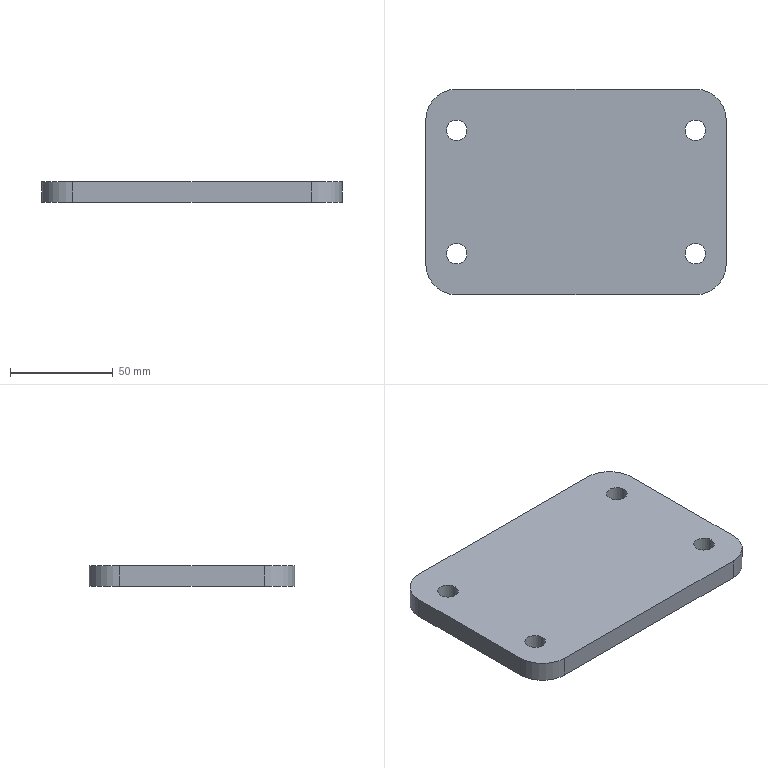Component | NX | BASE_100 | 1 solid | 14 faces | box 146 x 100 x 10 mm | volume 140927 mm3 | cylinder 8 | plane 6 | commonest cylinder face diameters 10 x4 30 x4
STEP:
#1=CARTESIAN_POINT('',(0.,0.,0.));
#2=DIRECTION('',(0.,0.,1.));
#3=DIRECTION('',(1.,0.,0.));
#4=AXIS2_PLACEMENT_3D('',#1,#2,#3);
#5=CARTESIAN_POINT('',(-73.,-35.,50.));
#6=VERTEX_POINT('',#5);
#7=CARTESIAN_POINT('',(-73.,35.,50.));
#8=VERTEX_POINT('',#7);
#9=CARTESIAN_POINT('',(-73.,-50.,50.));
#10=DIRECTION('',(0.,1.,0.));
#11=VECTOR('',#10,1.);
#12=LINE('',#9,#11);
#13=CARTESIAN_POINT('',(-73.,-50.,50.));
#14=DIRECTION('',(1.,0.,0.));
#15=DIRECTION('',(0.,0.,1.));
#16=AXIS2_PLACEMENT_3D('',#13,#14,#15);
#17=PLANE('',#16);
#18=CARTESIAN_POINT('',(0.,0.));
#19=DIRECTION('',(0.,-1.));
#20=VECTOR('',#19,1.);
#21=LINE('',#18,#20);
#22=(GEOMETRIC_REPRESENTATION_CONTEXT(2)PARAMETRIC_REPRESENTATION_CONTEXT()REPRESENTATION_CONTEXT('',''));
#23=DEFINITIONAL_REPRESENTATION('',(#21),#22);
#24=PCURVE('',#17,#23);
#25=CARTESIAN_POINT('',(-58.,30.,50.));
#26=DIRECTION('',(0.,0.,-1.));
#27=DIRECTION('',(1.,0.,0.));
#28=AXIS2_PLACEMENT_3D('',#25,#26,#27);
#29=PLANE('',#28);
#30=CARTESIAN_POINT('',(-15.,80.));
#31=DIRECTION('',(0.,-1.));
#32=VECTOR('',#31,1.);
#33=LINE('',#30,#32);
#34=(GEOMETRIC_REPRESENTATION_CONTEXT(2)PARAMETRIC_REPRESENTATION_CONTEXT()REPRESENTATION_CONTEXT('',''));
#35=DEFINITIONAL_REPRESENTATION('',(#33),#34);
#36=PCURVE('',#29,#35);
#37=SURFACE_CURVE('',#12,(#24,#36),.PCURVE_S1.);
#38=EDGE_CURVE('',#6,#8,#37,.T.);
#39=ORIENTED_EDGE('',*,*,#38,.F.);
#40=CARTESIAN_POINT('',(-73.,-35.,60.));
#41=VERTEX_POINT('',#40);
#42=CARTESIAN_POINT('',(-73.,-35.,50.));
#43=DIRECTION('',(0.,0.,1.));
#44=VECTOR('',#43,1.);
#45=LINE('',#42,#44);
#46=CARTESIAN_POINT('',(0.,-15.));
#47=DIRECTION('',(1.,0.));
#48=VECTOR('',#47,1.);
#49=LINE('',#46,#48);
#50=(GEOMETRIC_REPRESENTATION_CONTEXT(2)PARAMETRIC_REPRESENTATION_CONTEXT()REPRESENTATION_CONTEXT('',''));
#51=DEFINITIONAL_REPRESENTATION('',(#49),#50);
#52=PCURVE('',#17,#51);
#53=CARTESIAN_POINT('',(-58.,-35.,50.));
#54=DIRECTION('',(0.,0.,1.));
#55=DIRECTION('',(-1.,0.,0.));
#56=AXIS2_PLACEMENT_3D('',#53,#54,#55);
#57=CYLINDRICAL_SURFACE('',#56,15.);
#58=CARTESIAN_POINT('',(0.,0.));
#59=DIRECTION('',(0.,1.));
#60=VECTOR('',#59,1.);
#61=LINE('',#58,#60);
#62=(GEOMETRIC_REPRESENTATION_CONTEXT(2)PARAMETRIC_REPRESENTATION_CONTEXT()REPRESENTATION_CONTEXT('',''));
#63=DEFINITIONAL_REPRESENTATION('',(#61),#62);
#64=PCURVE('',#57,#63);
#65=SURFACE_CURVE('',#45,(#52,#64),.PCURVE_S1.);
#66=EDGE_CURVE('',#6,#41,#65,.T.);
#67=ORIENTED_EDGE('',*,*,#66,.T.);
#68=CARTESIAN_POINT('',(-73.,35.,60.));
#69=VERTEX_POINT('',#68);
#70=CARTESIAN_POINT('',(-73.,-50.,60.));
#71=DIRECTION('',(0.,1.,0.));
#72=VECTOR('',#71,1.);
#73=LINE('',#70,#72);
#74=CARTESIAN_POINT('',(10.,0.));
#75=DIRECTION('',(0.,-1.));
#76=VECTOR('',#75,1.);
#77=LINE('',#74,#76);
#78=(GEOMETRIC_REPRESENTATION_CONTEXT(2)PARAMETRIC_REPRESENTATION_CONTEXT()REPRESENTATION_CONTEXT('',''));
#79=DEFINITIONAL_REPRESENTATION('',(#77),#78);
#80=PCURVE('',#17,#79);
#81=CARTESIAN_POINT('',(-58.,30.,60.));
#82=DIRECTION('',(0.,0.,-1.));
#83=DIRECTION('',(1.,0.,0.));
#84=AXIS2_PLACEMENT_3D('',#81,#82,#83);
#85=PLANE('',#84);
#86=CARTESIAN_POINT('',(-15.,80.));
#87=DIRECTION('',(0.,-1.));
#88=VECTOR('',#87,1.);
#89=LINE('',#86,#88);
#90=(GEOMETRIC_REPRESENTATION_CONTEXT(2)PARAMETRIC_REPRESENTATION_CONTEXT()REPRESENTATION_CONTEXT('',''));
#91=DEFINITIONAL_REPRESENTATION('',(#89),#90);
#92=PCURVE('',#85,#91);
#93=SURFACE_CURVE('',#73,(#80,#92),.PCURVE_S1.);
#94=EDGE_CURVE('',#41,#69,#93,.T.);
#95=ORIENTED_EDGE('',*,*,#94,.T.);
#96=CARTESIAN_POINT('',(-73.,35.,50.));
#97=DIRECTION('',(0.,0.,-1.));
#98=VECTOR('',#97,1.);
#99=LINE('',#96,#98);
#100=CARTESIAN_POINT('',(0.,-85.));
#101=DIRECTION('',(-1.,0.));
#102=VECTOR('',#101,1.);
#103=LINE('',#100,#102);
#104=(GEOMETRIC_REPRESENTATION_CONTEXT(2)PARAMETRIC_REPRESENTATION_CONTEXT()REPRESENTATION_CONTEXT('',''));
#105=DEFINITIONAL_REPRESENTATION('',(#103),#104);
#106=PCURVE('',#17,#105);
#107=CARTESIAN_POINT('',(-58.,35.,50.));
#108=DIRECTION('',(0.,0.,1.));
#109=DIRECTION('',(-1.,0.,0.));
#110=AXIS2_PLACEMENT_3D('',#107,#108,#109);
#111=CYLINDRICAL_SURFACE('',#110,15.);
#112=CARTESIAN_POINT('',(6.283,0.));
#113=DIRECTION('',(0.,-1.));
#114=VECTOR('',#113,1.);
#115=LINE('',#112,#114);
#116=(GEOMETRIC_REPRESENTATION_CONTEXT(2)PARAMETRIC_REPRESENTATION_CONTEXT()REPRESENTATION_CONTEXT('',''));
#117=DEFINITIONAL_REPRESENTATION('',(#115),#116);
#118=PCURVE('',#111,#117);
#119=SURFACE_CURVE('',#99,(#106,#118),.PCURVE_S1.);
#120=EDGE_CURVE('',#69,#8,#119,.T.);
#121=ORIENTED_EDGE('',*,*,#120,.T.);
#122=EDGE_LOOP('',(#39,#67,#95,#121));
#123=FACE_BOUND('',#122,.T.);
#124=ADVANCED_FACE('',(#123),#17,.F.);
#125=CARTESIAN_POINT('',(-58.,50.,60.));
#126=VERTEX_POINT('',#125);
#127=CARTESIAN_POINT('',(58.,50.,60.));
#128=VERTEX_POINT('',#127);
#129=CARTESIAN_POINT('',(-73.,50.,60.));
#130=DIRECTION('',(1.,0.,0.));
#131=VECTOR('',#130,1.);
#132=LINE('',#129,#131);
#133=CARTESIAN_POINT('',(-73.,50.,50.));
#134=DIRECTION('',(0.,-1.,0.));
#135=DIRECTION('',(-1.,-0.,0.));
#136=AXIS2_PLACEMENT_3D('',#133,#134,#135);
#137=PLANE('',#136);
#138=CARTESIAN_POINT('',(0.,-10.));
#139=DIRECTION('',(-1.,0.));
#140=VECTOR('',#139,1.);
#141=LINE('',#138,#140);
#142=(GEOMETRIC_REPRESENTATION_CONTEXT(2)PARAMETRIC_REPRESENTATION_CONTEXT()REPRESENTATION_CONTEXT('',''));
#143=DEFINITIONAL_REPRESENTATION('',(#141),#142);
#144=PCURVE('',#137,#143);
#145=CARTESIAN_POINT('',(-15.,-20.));
#146=DIRECTION('',(1.,-0.));
#147=VECTOR('',#146,1.);
#148=LINE('',#145,#147);
#149=(GEOMETRIC_REPRESENTATION_CONTEXT(2)PARAMETRIC_REPRESENTATION_CONTEXT()REPRESENTATION_CONTEXT('',''));
#150=DEFINITIONAL_REPRESENTATION('',(#148),#149);
#151=PCURVE('',#85,#150);
#152=SURFACE_CURVE('',#132,(#144,#151),.PCURVE_S1.);
#153=EDGE_CURVE('',#126,#128,#152,.T.);
#154=ORIENTED_EDGE('',*,*,#153,.T.);
#155=CARTESIAN_POINT('',(58.,50.,50.));
#156=VERTEX_POINT('',#155);
#157=CARTESIAN_POINT('',(58.,50.,50.));
#158=DIRECTION('',(0.,0.,-1.));
#159=VECTOR('',#158,1.);
#160=LINE('',#157,#159);
#161=CARTESIAN_POINT('',(-131.,0.));
#162=DIRECTION('',(0.,1.));
#163=VECTOR('',#162,1.);
#164=LINE('',#161,#163);
#165=(GEOMETRIC_REPRESENTATION_CONTEXT(2)PARAMETRIC_REPRESENTATION_CONTEXT()REPRESENTATION_CONTEXT('',''));
#166=DEFINITIONAL_REPRESENTATION('',(#164),#165);
#167=PCURVE('',#137,#166);
#168=CARTESIAN_POINT('',(58.,35.,50.));
#169=DIRECTION('',(0.,0.,1.));
#170=DIRECTION('',(-1.,0.,0.));
#171=AXIS2_PLACEMENT_3D('',#168,#169,#170);
#172=CYLINDRICAL_SURFACE('',#171,15.);
#173=CARTESIAN_POINT('',(4.712,0.));
#174=DIRECTION('',(0.,-1.));
#175=VECTOR('',#174,1.);
#176=LINE('',#173,#175);
#177=(GEOMETRIC_REPRESENTATION_CONTEXT(2)PARAMETRIC_REPRESENTATION_CONTEXT()REPRESENTATION_CONTEXT('',''));
#178=DEFINITIONAL_REPRESENTATION('',(#176),#177);
#179=PCURVE('',#172,#178);
#180=SURFACE_CURVE('',#160,(#167,#179),.PCURVE_S1.);
#181=EDGE_CURVE('',#128,#156,#180,.T.);
#182=ORIENTED_EDGE('',*,*,#181,.T.);
#183=CARTESIAN_POINT('',(-58.,50.,50.));
#184=VERTEX_POINT('',#183);
#185=CARTESIAN_POINT('',(-73.,50.,50.));
#186=DIRECTION('',(1.,0.,0.));
#187=VECTOR('',#186,1.);
#188=LINE('',#185,#187);
#189=CARTESIAN_POINT('',(0.,0.));
#190=DIRECTION('',(-1.,0.));
#191=VECTOR('',#190,1.);
#192=LINE('',#189,#191);
#193=(GEOMETRIC_REPRESENTATION_CONTEXT(2)PARAMETRIC_REPRESENTATION_CONTEXT()REPRESENTATION_CONTEXT('',''));
#194=DEFINITIONAL_REPRESENTATION('',(#192),#193);
#195=PCURVE('',#137,#194);
#196=CARTESIAN_POINT('',(-15.,-20.));
#197=DIRECTION('',(1.,-0.));
#198=VECTOR('',#197,1.);
#199=LINE('',#196,#198);
#200=(GEOMETRIC_REPRESENTATION_CONTEXT(2)PARAMETRIC_REPRESENTATION_CONTEXT()REPRESENTATION_CONTEXT('',''));
#201=DEFINITIONAL_REPRESENTATION('',(#199),#200);
#202=PCURVE('',#29,#201);
#203=SURFACE_CURVE('',#188,(#195,#202),.PCURVE_S1.);
#204=EDGE_CURVE('',#184,#156,#203,.T.);
#205=ORIENTED_EDGE('',*,*,#204,.F.);
#206=CARTESIAN_POINT('',(-58.,50.,50.));
#207=DIRECTION('',(0.,0.,1.));
#208=VECTOR('',#207,1.);
#209=LINE('',#206,#208);
#210=CARTESIAN_POINT('',(-15.,0.));
#211=DIRECTION('',(0.,-1.));
#212=VECTOR('',#211,1.);
#213=LINE('',#210,#212);
#214=(GEOMETRIC_REPRESENTATION_CONTEXT(2)PARAMETRIC_REPRESENTATION_CONTEXT()REPRESENTATION_CONTEXT('',''));
#215=DEFINITIONAL_REPRESENTATION('',(#213),#214);
#216=PCURVE('',#137,#215);
#217=CARTESIAN_POINT('',(4.712,0.));
#218=DIRECTION('',(0.,1.));
#219=VECTOR('',#218,1.);
#220=LINE('',#217,#219);
#221=(GEOMETRIC_REPRESENTATION_CONTEXT(2)PARAMETRIC_REPRESENTATION_CONTEXT()REPRESENTATION_CONTEXT('',''));
#222=DEFINITIONAL_REPRESENTATION('',(#220),#221);
#223=PCURVE('',#111,#222);
#224=SURFACE_CURVE('',#209,(#216,#223),.PCURVE_S1.);
#225=EDGE_CURVE('',#184,#126,#224,.T.);
#226=ORIENTED_EDGE('',*,*,#225,.T.);
#227=EDGE_LOOP('',(#154,#182,#205,#226));
#228=FACE_BOUND('',#227,.T.);
#229=ADVANCED_FACE('',(#228),#137,.F.);
#230=CARTESIAN_POINT('',(73.,35.,60.));
#231=VERTEX_POINT('',#230);
#232=CARTESIAN_POINT('',(73.,-35.,60.));
#233=VERTEX_POINT('',#232);
#234=CARTESIAN_POINT('',(73.,50.,60.));
#235=DIRECTION('',(0.,-1.,0.));
#236=VECTOR('',#235,1.);
#237=LINE('',#234,#236);
#238=CARTESIAN_POINT('',(73.,50.,50.));
#239=DIRECTION('',(-1.,-0.,0.));
#240=DIRECTION('',(-0.,1.,0.));
#241=AXIS2_PLACEMENT_3D('',#238,#239,#240);
#242=PLANE('',#241);
#243=CARTESIAN_POINT('',(0.,-10.));
#244=DIRECTION('',(-1.,0.));
#245=VECTOR('',#244,1.);
#246=LINE('',#243,#245);
#247=(GEOMETRIC_REPRESENTATION_CONTEXT(2)PARAMETRIC_REPRESENTATION_CONTEXT()REPRESENTATION_CONTEXT('',''));
#248=DEFINITIONAL_REPRESENTATION('',(#246),#247);
#249=PCURVE('',#242,#248);
#250=CARTESIAN_POINT('',(131.,-20.));
#251=DIRECTION('',(0.,1.));
#252=VECTOR('',#251,1.);
#253=LINE('',#250,#252);
#254=(GEOMETRIC_REPRESENTATION_CONTEXT(2)PARAMETRIC_REPRESENTATION_CONTEXT()REPRESENTATION_CONTEXT('',''));
#255=DEFINITIONAL_REPRESENTATION('',(#253),#254);
#256=PCURVE('',#85,#255);
#257=SURFACE_CURVE('',#237,(#249,#256),.PCURVE_S1.);
#258=EDGE_CURVE('',#231,#233,#257,.T.);
#259=ORIENTED_EDGE('',*,*,#258,.T.);
#260=CARTESIAN_POINT('',(73.,-35.,50.));
#261=VERTEX_POINT('',#260);
#262=CARTESIAN_POINT('',(73.,-35.,50.));
#263=DIRECTION('',(0.,0.,-1.));
#264=VECTOR('',#263,1.);
#265=LINE('',#262,#264);
#266=CARTESIAN_POINT('',(-85.,0.));
#267=DIRECTION('',(0.,1.));
#268=VECTOR('',#267,1.);
#269=LINE('',#266,#268);
#270=(GEOMETRIC_REPRESENTATION_CONTEXT(2)PARAMETRIC_REPRESENTATION_CONTEXT()REPRESENTATION_CONTEXT('',''));
#271=DEFINITIONAL_REPRESENTATION('',(#269),#270);
#272=PCURVE('',#242,#271);
#273=CARTESIAN_POINT('',(58.,-35.,50.));
#274=DIRECTION('',(0.,0.,1.));
#275=DIRECTION('',(-1.,0.,0.));
#276=AXIS2_PLACEMENT_3D('',#273,#274,#275);
#277=CYLINDRICAL_SURFACE('',#276,15.);
#278=CARTESIAN_POINT('',(3.142,0.));
#279=DIRECTION('',(0.,-1.));
#280=VECTOR('',#279,1.);
#281=LINE('',#278,#280);
#282=(GEOMETRIC_REPRESENTATION_CONTEXT(2)PARAMETRIC_REPRESENTATION_CONTEXT()REPRESENTATION_CONTEXT('',''));
#283=DEFINITIONAL_REPRESENTATION('',(#281),#282);
#284=PCURVE('',#277,#283);
#285=SURFACE_CURVE('',#265,(#272,#284),.PCURVE_S1.);
#286=EDGE_CURVE('',#233,#261,#285,.T.);
#287=ORIENTED_EDGE('',*,*,#286,.T.);
#288=CARTESIAN_POINT('',(73.,35.,50.));
#289=VERTEX_POINT('',#288);
#290=CARTESIAN_POINT('',(73.,50.,50.));
#291=DIRECTION('',(0.,-1.,0.));
#292=VECTOR('',#291,1.);
#293=LINE('',#290,#292);
#294=CARTESIAN_POINT('',(0.,0.));
#295=DIRECTION('',(-1.,0.));
#296=VECTOR('',#295,1.);
#297=LINE('',#294,#296);
#298=(GEOMETRIC_REPRESENTATION_CONTEXT(2)PARAMETRIC_REPRESENTATION_CONTEXT()REPRESENTATION_CONTEXT('',''));
#299=DEFINITIONAL_REPRESENTATION('',(#297),#298);
#300=PCURVE('',#242,#299);
#301=CARTESIAN_POINT('',(131.,-20.));
#302=DIRECTION('',(0.,1.));
#303=VECTOR('',#302,1.);
#304=LINE('',#301,#303);
#305=(GEOMETRIC_REPRESENTATION_CONTEXT(2)PARAMETRIC_REPRESENTATION_CONTEXT()REPRESENTATION_CONTEXT('',''));
#306=DEFINITIONAL_REPRESENTATION('',(#304),#305);
#307=PCURVE('',#29,#306);
#308=SURFACE_CURVE('',#293,(#300,#307),.PCURVE_S1.);
#309=EDGE_CURVE('',#289,#261,#308,.T.);
#310=ORIENTED_EDGE('',*,*,#309,.F.);
#311=CARTESIAN_POINT('',(73.,35.,50.));
#312=DIRECTION('',(0.,0.,1.));
#313=VECTOR('',#312,1.);
#314=LINE('',#311,#313);
#315=CARTESIAN_POINT('',(-15.,0.));
#316=DIRECTION('',(0.,-1.));
#317=VECTOR('',#316,1.);
#318=LINE('',#315,#317);
#319=(GEOMETRIC_REPRESENTATION_CONTEXT(2)PARAMETRIC_REPRESENTATION_CONTEXT()REPRESENTATION_CONTEXT('',''));
#320=DEFINITIONAL_REPRESENTATION('',(#318),#319);
#321=PCURVE('',#242,#320);
#322=CARTESIAN_POINT('',(3.142,0.));
#323=DIRECTION('',(0.,1.));
#324=VECTOR('',#323,1.);
#325=LINE('',#322,#324);
#326=(GEOMETRIC_REPRESENTATION_CONTEXT(2)PARAMETRIC_REPRESENTATION_CONTEXT()REPRESENTATION_CONTEXT('',''));
#327=DEFINITIONAL_REPRESENTATION('',(#325),#326);
#328=PCURVE('',#172,#327);
#329=SURFACE_CURVE('',#314,(#321,#328),.PCURVE_S1.);
#330=EDGE_CURVE('',#289,#231,#329,.T.);
#331=ORIENTED_EDGE('',*,*,#330,.T.);
#332=EDGE_LOOP('',(#259,#287,#310,#331));
#333=FACE_BOUND('',#332,.T.);
#334=ADVANCED_FACE('',(#333),#242,.F.);
#335=CARTESIAN_POINT('',(63.,30.,50.));
#336=VERTEX_POINT('',#335);
#337=CARTESIAN_POINT('',(58.,30.,50.));
#338=DIRECTION('',(0.,0.,-1.));
#339=DIRECTION('',(1.,0.,0.));
#340=AXIS2_PLACEMENT_3D('',#337,#338,#339);
#341=CIRCLE('',#340,5.);
#342=CARTESIAN_POINT('',(58.,30.,50.));
#343=DIRECTION('',(0.,0.,1.));
#344=DIRECTION('',(-1.,0.,0.));
#345=AXIS2_PLACEMENT_3D('',#342,#343,#344);
#346=CYLINDRICAL_SURFACE('',#345,5.);
#347=CARTESIAN_POINT('',(9.425,0.));
#348=DIRECTION('',(-1.,0.));
#349=VECTOR('',#348,1.);
#350=LINE('',#347,#349);
#351=(GEOMETRIC_REPRESENTATION_CONTEXT(2)PARAMETRIC_REPRESENTATION_CONTEXT()REPRESENTATION_CONTEXT('',''));
#352=DEFINITIONAL_REPRESENTATION('',(#350),#351);
#353=PCURVE('',#346,#352);
#354=CARTESIAN_POINT('',(116.,0.));
#355=DIRECTION('',(1.,0.));
#356=AXIS2_PLACEMENT_2D('',#354,#355);
#357=CIRCLE('',#356,5.);
#358=(GEOMETRIC_REPRESENTATION_CONTEXT(2)PARAMETRIC_REPRESENTATION_CONTEXT()REPRESENTATION_CONTEXT('',''));
#359=DEFINITIONAL_REPRESENTATION('',(#357),#358);
#360=PCURVE('',#29,#359);
#361=SURFACE_CURVE('',#341,(#353,#360),.PCURVE_S1.);
#362=EDGE_CURVE('',#336,#336,#361,.T.);
#363=ORIENTED_EDGE('',*,*,#362,.F.);
#364=CARTESIAN_POINT('',(63.,30.,60.));
#365=VERTEX_POINT('',#364);
#366=CARTESIAN_POINT('',(63.,30.,50.));
#367=CARTESIAN_POINT('',(63.,30.,60.));
#368=B_SPLINE_CURVE_WITH_KNOTS('',1,(#366,#367),.UNSPECIFIED.,.F.,.F.,(2,2),(0.,10.),.PIECEWISE_BEZIER_KNOTS.);
#369=CARTESIAN_POINT('',(9.425,0.));
#370=DIRECTION('',(0.,1.));
#371=VECTOR('',#370,1.);
#372=LINE('',#369,#371);
#373=(GEOMETRIC_REPRESENTATION_CONTEXT(2)PARAMETRIC_REPRESENTATION_CONTEXT()REPRESENTATION_CONTEXT('',''));
#374=DEFINITIONAL_REPRESENTATION('',(#372),#373);
#375=PCURVE('',#346,#374);
#376=CARTESIAN_POINT('',(3.142,0.));
#377=DIRECTION('',(0.,1.));
#378=VECTOR('',#377,1.);
#379=LINE('',#376,#378);
#380=(GEOMETRIC_REPRESENTATION_CONTEXT(2)PARAMETRIC_REPRESENTATION_CONTEXT()REPRESENTATION_CONTEXT('',''));
#381=DEFINITIONAL_REPRESENTATION('',(#379),#380);
#382=PCURVE('',#346,#381);
#383=SEAM_CURVE('',#368,(#375,#382),.PCURVE_S1.);
#384=EDGE_CURVE('',#336,#365,#383,.T.);
#385=ORIENTED_EDGE('',*,*,#384,.T.);
#386=CARTESIAN_POINT('',(58.,30.,60.));
#387=DIRECTION('',(0.,0.,-1.));
#388=DIRECTION('',(1.,0.,0.));
#389=AXIS2_PLACEMENT_3D('',#386,#387,#388);
#390=CIRCLE('',#389,5.);
#391=CARTESIAN_POINT('',(9.425,10.));
#392=DIRECTION('',(-1.,0.));
#393=VECTOR('',#392,1.);
#394=LINE('',#391,#393);
#395=(GEOMETRIC_REPRESENTATION_CONTEXT(2)PARAMETRIC_REPRESENTATION_CONTEXT()REPRESENTATION_CONTEXT('',''));
#396=DEFINITIONAL_REPRESENTATION('',(#394),#395);
#397=PCURVE('',#346,#396);
#398=CARTESIAN_POINT('',(116.,0.));
#399=DIRECTION('',(1.,0.));
#400=AXIS2_PLACEMENT_2D('',#398,#399);
#401=CIRCLE('',#400,5.);
#402=(GEOMETRIC_REPRESENTATION_CONTEXT(2)PARAMETRIC_REPRESENTATION_CONTEXT()REPRESENTATION_CONTEXT('',''));
#403=DEFINITIONAL_REPRESENTATION('',(#401),#402);
#404=PCURVE('',#85,#403);
#405=SURFACE_CURVE('',#390,(#397,#404),.PCURVE_S1.);
#406=EDGE_CURVE('',#365,#365,#405,.T.);
#407=ORIENTED_EDGE('',*,*,#406,.T.);
#408=ORIENTED_EDGE('',*,*,#384,.F.);
#409=EDGE_LOOP('',(#363,#385,#407,#408));
#410=FACE_BOUND('',#409,.F.);
#411=ADVANCED_FACE('',(#410),#346,.F.);
#412=CARTESIAN_POINT('',(-53.,-30.,50.));
#413=VERTEX_POINT('',#412);
#414=CARTESIAN_POINT('',(-58.,-30.,50.));
#415=DIRECTION('',(0.,0.,-1.));
#416=DIRECTION('',(1.,0.,0.));
#417=AXIS2_PLACEMENT_3D('',#414,#415,#416);
#418=CIRCLE('',#417,5.);
#419=CARTESIAN_POINT('',(-58.,-30.,50.));
#420=DIRECTION('',(0.,0.,1.));
#421=DIRECTION('',(-1.,0.,0.));
#422=AXIS2_PLACEMENT_3D('',#419,#420,#421);
#423=CYLINDRICAL_SURFACE('',#422,5.);
#424=CARTESIAN_POINT('',(9.425,0.));
#425=DIRECTION('',(-1.,0.));
#426=VECTOR('',#425,1.);
#427=LINE('',#424,#426);
#428=(GEOMETRIC_REPRESENTATION_CONTEXT(2)PARAMETRIC_REPRESENTATION_CONTEXT()REPRESENTATION_CONTEXT('',''));
#429=DEFINITIONAL_REPRESENTATION('',(#427),#428);
#430=PCURVE('',#423,#429);
#431=CARTESIAN_POINT('',(0.,60.));
#432=DIRECTION('',(1.,0.));
#433=AXIS2_PLACEMENT_2D('',#431,#432);
#434=CIRCLE('',#433,5.);
#435=(GEOMETRIC_REPRESENTATION_CONTEXT(2)PARAMETRIC_REPRESENTATION_CONTEXT()REPRESENTATION_CONTEXT('',''));
#436=DEFINITIONAL_REPRESENTATION('',(#434),#435);
#437=PCURVE('',#29,#436);
#438=SURFACE_CURVE('',#418,(#430,#437),.PCURVE_S1.);
#439=EDGE_CURVE('',#413,#413,#438,.T.);
#440=ORIENTED_EDGE('',*,*,#439,.F.);
#441=CARTESIAN_POINT('',(-53.,-30.,60.));
#442=VERTEX_POINT('',#441);
#443=CARTESIAN_POINT('',(-53.,-30.,50.));
#444=CARTESIAN_POINT('',(-53.,-30.,60.));
#445=B_SPLINE_CURVE_WITH_KNOTS('',1,(#443,#444),.UNSPECIFIED.,.F.,.F.,(2,2),(0.,10.),.PIECEWISE_BEZIER_KNOTS.);
#446=CARTESIAN_POINT('',(9.425,0.));
#447=DIRECTION('',(0.,1.));
#448=VECTOR('',#447,1.);
#449=LINE('',#446,#448);
#450=(GEOMETRIC_REPRESENTATION_CONTEXT(2)PARAMETRIC_REPRESENTATION_CONTEXT()REPRESENTATION_CONTEXT('',''));
#451=DEFINITIONAL_REPRESENTATION('',(#449),#450);
#452=PCURVE('',#423,#451);
#453=CARTESIAN_POINT('',(3.142,0.));
#454=DIRECTION('',(0.,1.));
#455=VECTOR('',#454,1.);
#456=LINE('',#453,#455);
#457=(GEOMETRIC_REPRESENTATION_CONTEXT(2)PARAMETRIC_REPRESENTATION_CONTEXT()REPRESENTATION_CONTEXT('',''));
#458=DEFINITIONAL_REPRESENTATION('',(#456),#457);
#459=PCURVE('',#423,#458);
#460=SEAM_CURVE('',#445,(#452,#459),.PCURVE_S1.);
#461=EDGE_CURVE('',#413,#442,#460,.T.);
#462=ORIENTED_EDGE('',*,*,#461,.T.);
#463=CARTESIAN_POINT('',(-58.,-30.,60.));
#464=DIRECTION('',(0.,0.,-1.));
#465=DIRECTION('',(1.,0.,0.));
#466=AXIS2_PLACEMENT_3D('',#463,#464,#465);
#467=CIRCLE('',#466,5.);
#468=CARTESIAN_POINT('',(9.425,10.));
#469=DIRECTION('',(-1.,0.));
#470=VECTOR('',#469,1.);
#471=LINE('',#468,#470);
#472=(GEOMETRIC_REPRESENTATION_CONTEXT(2)PARAMETRIC_REPRESENTATION_CONTEXT()REPRESENTATION_CONTEXT('',''));
#473=DEFINITIONAL_REPRESENTATION('',(#471),#472);
#474=PCURVE('',#423,#473);
#475=CARTESIAN_POINT('',(0.,60.));
#476=DIRECTION('',(1.,0.));
#477=AXIS2_PLACEMENT_2D('',#475,#476);
#478=CIRCLE('',#477,5.);
#479=(GEOMETRIC_REPRESENTATION_CONTEXT(2)PARAMETRIC_REPRESENTATION_CONTEXT()REPRESENTATION_CONTEXT('',''));
#480=DEFINITIONAL_REPRESENTATION('',(#478),#479);
#481=PCURVE('',#85,#480);
#482=SURFACE_CURVE('',#467,(#474,#481),.PCURVE_S1.);
#483=EDGE_CURVE('',#442,#442,#482,.T.);
#484=ORIENTED_EDGE('',*,*,#483,.T.);
#485=ORIENTED_EDGE('',*,*,#461,.F.);
#486=EDGE_LOOP('',(#440,#462,#484,#485));
#487=FACE_BOUND('',#486,.F.);
#488=ADVANCED_FACE('',(#487),#423,.F.);
#489=CARTESIAN_POINT('',(-53.,30.,50.));
#490=VERTEX_POINT('',#489);
#491=CARTESIAN_POINT('',(-58.,30.,50.));
#492=DIRECTION('',(0.,0.,-1.));
#493=DIRECTION('',(1.,0.,0.));
#494=AXIS2_PLACEMENT_3D('',#491,#492,#493);
#495=CIRCLE('',#494,5.);
#496=CARTESIAN_POINT('',(-58.,30.,50.));
#497=DIRECTION('',(0.,0.,1.));
#498=DIRECTION('',(-1.,0.,0.));
#499=AXIS2_PLACEMENT_3D('',#496,#497,#498);
#500=CYLINDRICAL_SURFACE('',#499,5.);
#501=CARTESIAN_POINT('',(9.425,0.));
#502=DIRECTION('',(-1.,0.));
#503=VECTOR('',#502,1.);
#504=LINE('',#501,#503);
#505=(GEOMETRIC_REPRESENTATION_CONTEXT(2)PARAMETRIC_REPRESENTATION_CONTEXT()REPRESENTATION_CONTEXT('',''));
#506=DEFINITIONAL_REPRESENTATION('',(#504),#505);
#507=PCURVE('',#500,#506);
#508=CARTESIAN_POINT('',(0.,0.));
#509=DIRECTION('',(1.,0.));
#510=AXIS2_PLACEMENT_2D('',#508,#509);
#511=CIRCLE('',#510,5.);
#512=(GEOMETRIC_REPRESENTATION_CONTEXT(2)PARAMETRIC_REPRESENTATION_CONTEXT()REPRESENTATION_CONTEXT('',''));
#513=DEFINITIONAL_REPRESENTATION('',(#511),#512);
#514=PCURVE('',#29,#513);
#515=SURFACE_CURVE('',#495,(#507,#514),.PCURVE_S1.);
#516=EDGE_CURVE('',#490,#490,#515,.T.);
#517=ORIENTED_EDGE('',*,*,#516,.F.);
#518=CARTESIAN_POINT('',(-53.,30.,60.));
#519=VERTEX_POINT('',#518);
#520=CARTESIAN_POINT('',(-53.,30.,50.));
#521=CARTESIAN_POINT('',(-53.,30.,60.));
#522=B_SPLINE_CURVE_WITH_KNOTS('',1,(#520,#521),.UNSPECIFIED.,.F.,.F.,(2,2),(0.,10.),.PIECEWISE_BEZIER_KNOTS.);
#523=CARTESIAN_POINT('',(9.425,0.));
#524=DIRECTION('',(0.,1.));
#525=VECTOR('',#524,1.);
#526=LINE('',#523,#525);
#527=(GEOMETRIC_REPRESENTATION_CONTEXT(2)PARAMETRIC_REPRESENTATION_CONTEXT()REPRESENTATION_CONTEXT('',''));
#528=DEFINITIONAL_REPRESENTATION('',(#526),#527);
#529=PCURVE('',#500,#528);
#530=CARTESIAN_POINT('',(3.142,0.));
#531=DIRECTION('',(0.,1.));
#532=VECTOR('',#531,1.);
#533=LINE('',#530,#532);
#534=(GEOMETRIC_REPRESENTATION_CONTEXT(2)PARAMETRIC_REPRESENTATION_CONTEXT()REPRESENTATION_CONTEXT('',''));
#535=DEFINITIONAL_REPRESENTATION('',(#533),#534);
#536=PCURVE('',#500,#535);
#537=SEAM_CURVE('',#522,(#529,#536),.PCURVE_S1.);
#538=EDGE_CURVE('',#490,#519,#537,.T.);
#539=ORIENTED_EDGE('',*,*,#538,.T.);
#540=CARTESIAN_POINT('',(-58.,30.,60.));
#541=DIRECTION('',(0.,0.,-1.));
#542=DIRECTION('',(1.,0.,0.));
#543=AXIS2_PLACEMENT_3D('',#540,#541,#542);
#544=CIRCLE('',#543,5.);
#545=CARTESIAN_POINT('',(9.425,10.));
#546=DIRECTION('',(-1.,0.));
#547=VECTOR('',#546,1.);
#548=LINE('',#545,#547);
#549=(GEOMETRIC_REPRESENTATION_CONTEXT(2)PARAMETRIC_REPRESENTATION_CONTEXT()REPRESENTATION_CONTEXT('',''));
#550=DEFINITIONAL_REPRESENTATION('',(#548),#549);
#551=PCURVE('',#500,#550);
#552=CARTESIAN_POINT('',(0.,0.));
#553=DIRECTION('',(1.,0.));
#554=AXIS2_PLACEMENT_2D('',#552,#553);
#555=CIRCLE('',#554,5.);
#556=(GEOMETRIC_REPRESENTATION_CONTEXT(2)PARAMETRIC_REPRESENTATION_CONTEXT()REPRESENTATION_CONTEXT('',''));
#557=DEFINITIONAL_REPRESENTATION('',(#555),#556);
#558=PCURVE('',#85,#557);
#559=SURFACE_CURVE('',#544,(#551,#558),.PCURVE_S1.);
#560=EDGE_CURVE('',#519,#519,#559,.T.);
#561=ORIENTED_EDGE('',*,*,#560,.T.);
#562=ORIENTED_EDGE('',*,*,#538,.F.);
#563=EDGE_LOOP('',(#517,#539,#561,#562));
#564=FACE_BOUND('',#563,.F.);
#565=ADVANCED_FACE('',(#564),#500,.F.);
#566=CARTESIAN_POINT('',(58.,-50.,60.));
#567=VERTEX_POINT('',#566);
#568=CARTESIAN_POINT('',(-58.,-50.,60.));
#569=VERTEX_POINT('',#568);
#570=CARTESIAN_POINT('',(73.,-50.,60.));
#571=DIRECTION('',(-1.,0.,0.));
#572=VECTOR('',#571,1.);
#573=LINE('',#570,#572);
#574=CARTESIAN_POINT('',(73.,-50.,50.));
#575=DIRECTION('',(0.,1.,0.));
#576=DIRECTION('',(1.,-0.,0.));
#577=AXIS2_PLACEMENT_3D('',#574,#575,#576);
#578=PLANE('',#577);
#579=CARTESIAN_POINT('',(0.,-10.));
#580=DIRECTION('',(-1.,0.));
#581=VECTOR('',#580,1.);
#582=LINE('',#579,#581);
#583=(GEOMETRIC_REPRESENTATION_CONTEXT(2)PARAMETRIC_REPRESENTATION_CONTEXT()REPRESENTATION_CONTEXT('',''));
#584=DEFINITIONAL_REPRESENTATION('',(#582),#583);
#585=PCURVE('',#578,#584);
#586=CARTESIAN_POINT('',(131.,80.));
#587=DIRECTION('',(-1.,-0.));
#588=VECTOR('',#587,1.);
#589=LINE('',#586,#588);
#590=(GEOMETRIC_REPRESENTATION_CONTEXT(2)PARAMETRIC_REPRESENTATION_CONTEXT()REPRESENTATION_CONTEXT('',''));
#591=DEFINITIONAL_REPRESENTATION('',(#589),#590);
#592=PCURVE('',#85,#591);
#593=SURFACE_CURVE('',#573,(#585,#592),.PCURVE_S1.);
#594=EDGE_CURVE('',#567,#569,#593,.T.);
#595=ORIENTED_EDGE('',*,*,#594,.T.);
#596=CARTESIAN_POINT('',(-58.,-50.,50.));
#597=VERTEX_POINT('',#596);
#598=CARTESIAN_POINT('',(-58.,-50.,50.));
#599=DIRECTION('',(0.,0.,-1.));
#600=VECTOR('',#599,1.);
#601=LINE('',#598,#600);
#602=CARTESIAN_POINT('',(-131.,0.));
#603=DIRECTION('',(0.,1.));
#604=VECTOR('',#603,1.);
#605=LINE('',#602,#604);
#606=(GEOMETRIC_REPRESENTATION_CONTEXT(2)PARAMETRIC_REPRESENTATION_CONTEXT()REPRESENTATION_CONTEXT('',''));
#607=DEFINITIONAL_REPRESENTATION('',(#605),#606);
#608=PCURVE('',#578,#607);
#609=CARTESIAN_POINT('',(1.571,0.));
#610=DIRECTION('',(0.,-1.));
#611=VECTOR('',#610,1.);
#612=LINE('',#609,#611);
#613=(GEOMETRIC_REPRESENTATION_CONTEXT(2)PARAMETRIC_REPRESENTATION_CONTEXT()REPRESENTATION_CONTEXT('',''));
#614=DEFINITIONAL_REPRESENTATION('',(#612),#613);
#615=PCURVE('',#57,#614);
#616=SURFACE_CURVE('',#601,(#608,#615),.PCURVE_S1.);
#617=EDGE_CURVE('',#569,#597,#616,.T.);
#618=ORIENTED_EDGE('',*,*,#617,.T.);
#619=CARTESIAN_POINT('',(58.,-50.,50.));
#620=VERTEX_POINT('',#619);
#621=CARTESIAN_POINT('',(73.,-50.,50.));
#622=DIRECTION('',(-1.,0.,0.));
#623=VECTOR('',#622,1.);
#624=LINE('',#621,#623);
#625=CARTESIAN_POINT('',(0.,0.));
#626=DIRECTION('',(-1.,0.));
#627=VECTOR('',#626,1.);
#628=LINE('',#625,#627);
#629=(GEOMETRIC_REPRESENTATION_CONTEXT(2)PARAMETRIC_REPRESENTATION_CONTEXT()REPRESENTATION_CONTEXT('',''));
#630=DEFINITIONAL_REPRESENTATION('',(#628),#629);
#631=PCURVE('',#578,#630);
#632=CARTESIAN_POINT('',(131.,80.));
#633=DIRECTION('',(-1.,-0.));
#634=VECTOR('',#633,1.);
#635=LINE('',#632,#634);
#636=(GEOMETRIC_REPRESENTATION_CONTEXT(2)PARAMETRIC_REPRESENTATION_CONTEXT()REPRESENTATION_CONTEXT('',''));
#637=DEFINITIONAL_REPRESENTATION('',(#635),#636);
#638=PCURVE('',#29,#637);
#639=SURFACE_CURVE('',#624,(#631,#638),.PCURVE_S1.);
#640=EDGE_CURVE('',#620,#597,#639,.T.);
#641=ORIENTED_EDGE('',*,*,#640,.F.);
#642=CARTESIAN_POINT('',(58.,-50.,50.));
#643=DIRECTION('',(0.,0.,1.));
#644=VECTOR('',#643,1.);
#645=LINE('',#642,#644);
#646=CARTESIAN_POINT('',(-15.,0.));
#647=DIRECTION('',(0.,-1.));
#648=VECTOR('',#647,1.);
#649=LINE('',#646,#648);
#650=(GEOMETRIC_REPRESENTATION_CONTEXT(2)PARAMETRIC_REPRESENTATION_CONTEXT()REPRESENTATION_CONTEXT('',''));
#651=DEFINITIONAL_REPRESENTATION('',(#649),#650);
#652=PCURVE('',#578,#651);
#653=CARTESIAN_POINT('',(1.571,0.));
#654=DIRECTION('',(0.,1.));
#655=VECTOR('',#654,1.);
#656=LINE('',#653,#655);
#657=(GEOMETRIC_REPRESENTATION_CONTEXT(2)PARAMETRIC_REPRESENTATION_CONTEXT()REPRESENTATION_CONTEXT('',''));
#658=DEFINITIONAL_REPRESENTATION('',(#656),#657);
#659=PCURVE('',#277,#658);
#660=SURFACE_CURVE('',#645,(#652,#659),.PCURVE_S1.);
#661=EDGE_CURVE('',#620,#567,#660,.T.);
#662=ORIENTED_EDGE('',*,*,#661,.T.);
#663=EDGE_LOOP('',(#595,#618,#641,#662));
#664=FACE_BOUND('',#663,.T.);
#665=ADVANCED_FACE('',(#664),#578,.F.);
#666=CARTESIAN_POINT('',(63.,-30.,50.));
#667=VERTEX_POINT('',#666);
#668=CARTESIAN_POINT('',(58.,-30.,50.));
#669=DIRECTION('',(0.,0.,-1.));
#670=DIRECTION('',(1.,0.,0.));
#671=AXIS2_PLACEMENT_3D('',#668,#669,#670);
#672=CIRCLE('',#671,5.);
#673=CARTESIAN_POINT('',(58.,-30.,50.));
#674=DIRECTION('',(0.,0.,1.));
#675=DIRECTION('',(-1.,0.,0.));
#676=AXIS2_PLACEMENT_3D('',#673,#674,#675);
#677=CYLINDRICAL_SURFACE('',#676,5.);
#678=CARTESIAN_POINT('',(9.425,0.));
#679=DIRECTION('',(-1.,0.));
#680=VECTOR('',#679,1.);
#681=LINE('',#678,#680);
#682=(GEOMETRIC_REPRESENTATION_CONTEXT(2)PARAMETRIC_REPRESENTATION_CONTEXT()REPRESENTATION_CONTEXT('',''));
#683=DEFINITIONAL_REPRESENTATION('',(#681),#682);
#684=PCURVE('',#677,#683);
#685=CARTESIAN_POINT('',(116.,60.));
#686=DIRECTION('',(1.,0.));
#687=AXIS2_PLACEMENT_2D('',#685,#686);
#688=CIRCLE('',#687,5.);
#689=(GEOMETRIC_REPRESENTATION_CONTEXT(2)PARAMETRIC_REPRESENTATION_CONTEXT()REPRESENTATION_CONTEXT('',''));
#690=DEFINITIONAL_REPRESENTATION('',(#688),#689);
#691=PCURVE('',#29,#690);
#692=SURFACE_CURVE('',#672,(#684,#691),.PCURVE_S1.);
#693=EDGE_CURVE('',#667,#667,#692,.T.);
#694=ORIENTED_EDGE('',*,*,#693,.F.);
#695=CARTESIAN_POINT('',(63.,-30.,60.));
#696=VERTEX_POINT('',#695);
#697=CARTESIAN_POINT('',(63.,-30.,50.));
#698=CARTESIAN_POINT('',(63.,-30.,60.));
#699=B_SPLINE_CURVE_WITH_KNOTS('',1,(#697,#698),.UNSPECIFIED.,.F.,.F.,(2,2),(0.,10.),.PIECEWISE_BEZIER_KNOTS.);
#700=CARTESIAN_POINT('',(9.425,0.));
#701=DIRECTION('',(0.,1.));
#702=VECTOR('',#701,1.);
#703=LINE('',#700,#702);
#704=(GEOMETRIC_REPRESENTATION_CONTEXT(2)PARAMETRIC_REPRESENTATION_CONTEXT()REPRESENTATION_CONTEXT('',''));
#705=DEFINITIONAL_REPRESENTATION('',(#703),#704);
#706=PCURVE('',#677,#705);
#707=CARTESIAN_POINT('',(3.142,0.));
#708=DIRECTION('',(0.,1.));
#709=VECTOR('',#708,1.);
#710=LINE('',#707,#709);
#711=(GEOMETRIC_REPRESENTATION_CONTEXT(2)PARAMETRIC_REPRESENTATION_CONTEXT()REPRESENTATION_CONTEXT('',''));
#712=DEFINITIONAL_REPRESENTATION('',(#710),#711);
#713=PCURVE('',#677,#712);
#714=SEAM_CURVE('',#699,(#706,#713),.PCURVE_S1.);
#715=EDGE_CURVE('',#667,#696,#714,.T.);
#716=ORIENTED_EDGE('',*,*,#715,.T.);
#717=CARTESIAN_POINT('',(58.,-30.,60.));
#718=DIRECTION('',(0.,0.,-1.));
#719=DIRECTION('',(1.,0.,0.));
#720=AXIS2_PLACEMENT_3D('',#717,#718,#719);
#721=CIRCLE('',#720,5.);
#722=CARTESIAN_POINT('',(9.425,10.));
#723=DIRECTION('',(-1.,0.));
#724=VECTOR('',#723,1.);
#725=LINE('',#722,#724);
#726=(GEOMETRIC_REPRESENTATION_CONTEXT(2)PARAMETRIC_REPRESENTATION_CONTEXT()REPRESENTATION_CONTEXT('',''));
#727=DEFINITIONAL_REPRESENTATION('',(#725),#726);
#728=PCURVE('',#677,#727);
#729=CARTESIAN_POINT('',(116.,60.));
#730=DIRECTION('',(1.,0.));
#731=AXIS2_PLACEMENT_2D('',#729,#730);
#732=CIRCLE('',#731,5.);
#733=(GEOMETRIC_REPRESENTATION_CONTEXT(2)PARAMETRIC_REPRESENTATION_CONTEXT()REPRESENTATION_CONTEXT('',''));
#734=DEFINITIONAL_REPRESENTATION('',(#732),#733);
#735=PCURVE('',#85,#734);
#736=SURFACE_CURVE('',#721,(#728,#735),.PCURVE_S1.);
#737=EDGE_CURVE('',#696,#696,#736,.T.);
#738=ORIENTED_EDGE('',*,*,#737,.T.);
#739=ORIENTED_EDGE('',*,*,#715,.F.);
#740=EDGE_LOOP('',(#694,#716,#738,#739));
#741=FACE_BOUND('',#740,.F.);
#742=ADVANCED_FACE('',(#741),#677,.F.);
#743=ORIENTED_EDGE('',*,*,#640,.T.);
#744=CARTESIAN_POINT('',(-58.,-35.,50.));
#745=DIRECTION('',(0.,0.,-1.));
#746=DIRECTION('',(1.,0.,0.));
#747=AXIS2_PLACEMENT_3D('',#744,#745,#746);
#748=CIRCLE('',#747,15.);
#749=CARTESIAN_POINT('',(0.,65.));
#750=DIRECTION('',(1.,0.));
#751=AXIS2_PLACEMENT_2D('',#749,#750);
#752=CIRCLE('',#751,15.);
#753=(GEOMETRIC_REPRESENTATION_CONTEXT(2)PARAMETRIC_REPRESENTATION_CONTEXT()REPRESENTATION_CONTEXT('',''));
#754=DEFINITIONAL_REPRESENTATION('',(#752),#753);
#755=PCURVE('',#29,#754);
#756=CARTESIAN_POINT('',(3.142,0.));
#757=DIRECTION('',(-1.,0.));
#758=VECTOR('',#757,1.);
#759=LINE('',#756,#758);
#760=(GEOMETRIC_REPRESENTATION_CONTEXT(2)PARAMETRIC_REPRESENTATION_CONTEXT()REPRESENTATION_CONTEXT('',''));
#761=DEFINITIONAL_REPRESENTATION('',(#759),#760);
#762=PCURVE('',#57,#761);
#763=SURFACE_CURVE('',#748,(#755,#762),.PCURVE_S1.);
#764=EDGE_CURVE('',#597,#6,#763,.T.);
#765=ORIENTED_EDGE('',*,*,#764,.T.);
#766=ORIENTED_EDGE('',*,*,#38,.T.);
#767=CARTESIAN_POINT('',(-58.,35.,50.));
#768=DIRECTION('',(0.,0.,-1.));
#769=DIRECTION('',(1.,0.,0.));
#770=AXIS2_PLACEMENT_3D('',#767,#768,#769);
#771=CIRCLE('',#770,15.);
#772=CARTESIAN_POINT('',(0.,-5.));
#773=DIRECTION('',(1.,0.));
#774=AXIS2_PLACEMENT_2D('',#772,#773);
#775=CIRCLE('',#774,15.);
#776=(GEOMETRIC_REPRESENTATION_CONTEXT(2)PARAMETRIC_REPRESENTATION_CONTEXT()REPRESENTATION_CONTEXT('',''));
#777=DEFINITIONAL_REPRESENTATION('',(#775),#776);
#778=PCURVE('',#29,#777);
#779=CARTESIAN_POINT('',(9.425,0.));
#780=DIRECTION('',(-1.,0.));
#781=VECTOR('',#780,1.);
#782=LINE('',#779,#781);
#783=(GEOMETRIC_REPRESENTATION_CONTEXT(2)PARAMETRIC_REPRESENTATION_CONTEXT()REPRESENTATION_CONTEXT('',''));
#784=DEFINITIONAL_REPRESENTATION('',(#782),#783);
#785=PCURVE('',#111,#784);
#786=SURFACE_CURVE('',#771,(#778,#785),.PCURVE_S1.);
#787=EDGE_CURVE('',#8,#184,#786,.T.);
#788=ORIENTED_EDGE('',*,*,#787,.T.);
#789=ORIENTED_EDGE('',*,*,#204,.T.);
#790=CARTESIAN_POINT('',(58.,35.,50.));
#791=DIRECTION('',(0.,0.,-1.));
#792=DIRECTION('',(1.,0.,0.));
#793=AXIS2_PLACEMENT_3D('',#790,#791,#792);
#794=CIRCLE('',#793,15.);
#795=CARTESIAN_POINT('',(116.,-5.));
#796=DIRECTION('',(1.,0.));
#797=AXIS2_PLACEMENT_2D('',#795,#796);
#798=CIRCLE('',#797,15.);
#799=(GEOMETRIC_REPRESENTATION_CONTEXT(2)PARAMETRIC_REPRESENTATION_CONTEXT()REPRESENTATION_CONTEXT('',''));
#800=DEFINITIONAL_REPRESENTATION('',(#798),#799);
#801=PCURVE('',#29,#800);
#802=CARTESIAN_POINT('',(9.425,0.));
#803=DIRECTION('',(-1.,0.));
#804=VECTOR('',#803,1.);
#805=LINE('',#802,#804);
#806=(GEOMETRIC_REPRESENTATION_CONTEXT(2)PARAMETRIC_REPRESENTATION_CONTEXT()REPRESENTATION_CONTEXT('',''));
#807=DEFINITIONAL_REPRESENTATION('',(#805),#806);
#808=PCURVE('',#172,#807);
#809=SURFACE_CURVE('',#794,(#801,#808),.PCURVE_S1.);
#810=EDGE_CURVE('',#156,#289,#809,.T.);
#811=ORIENTED_EDGE('',*,*,#810,.T.);
#812=ORIENTED_EDGE('',*,*,#309,.T.);
#813=CARTESIAN_POINT('',(58.,-35.,50.));
#814=DIRECTION('',(0.,0.,-1.));
#815=DIRECTION('',(1.,0.,0.));
#816=AXIS2_PLACEMENT_3D('',#813,#814,#815);
#817=CIRCLE('',#816,15.);
#818=CARTESIAN_POINT('',(116.,65.));
#819=DIRECTION('',(1.,0.));
#820=AXIS2_PLACEMENT_2D('',#818,#819);
#821=CIRCLE('',#820,15.);
#822=(GEOMETRIC_REPRESENTATION_CONTEXT(2)PARAMETRIC_REPRESENTATION_CONTEXT()REPRESENTATION_CONTEXT('',''));
#823=DEFINITIONAL_REPRESENTATION('',(#821),#822);
#824=PCURVE('',#29,#823);
#825=CARTESIAN_POINT('',(3.142,0.));
#826=DIRECTION('',(-1.,0.));
#827=VECTOR('',#826,1.);
#828=LINE('',#825,#827);
#829=(GEOMETRIC_REPRESENTATION_CONTEXT(2)PARAMETRIC_REPRESENTATION_CONTEXT()REPRESENTATION_CONTEXT('',''));
#830=DEFINITIONAL_REPRESENTATION('',(#828),#829);
#831=PCURVE('',#277,#830);
#832=SURFACE_CURVE('',#817,(#824,#831),.PCURVE_S1.);
#833=EDGE_CURVE('',#261,#620,#832,.T.);
#834=ORIENTED_EDGE('',*,*,#833,.T.);
#835=EDGE_LOOP('',(#743,#765,#766,#788,#789,#811,#812,#834));
#836=FACE_BOUND('',#835,.T.);
#837=ORIENTED_EDGE('',*,*,#516,.F.);
#838=EDGE_LOOP('',(#837));
#839=FACE_BOUND('',#838,.T.);
#840=ORIENTED_EDGE('',*,*,#439,.F.);
#841=EDGE_LOOP('',(#840));
#842=FACE_BOUND('',#841,.T.);
#843=ORIENTED_EDGE('',*,*,#362,.F.);
#844=EDGE_LOOP('',(#843));
#845=FACE_BOUND('',#844,.T.);
#846=ORIENTED_EDGE('',*,*,#693,.F.);
#847=EDGE_LOOP('',(#846));
#848=FACE_BOUND('',#847,.T.);
#849=ADVANCED_FACE('',(#836,#839,#842,#845,#848),#29,.T.);
#850=ORIENTED_EDGE('',*,*,#94,.F.);
#851=CARTESIAN_POINT('',(-58.,-35.,60.));
#852=DIRECTION('',(0.,0.,1.));
#853=DIRECTION('',(1.,0.,0.));
#854=AXIS2_PLACEMENT_3D('',#851,#852,#853);
#855=CIRCLE('',#854,15.);
#856=CARTESIAN_POINT('',(15.,65.));
#857=CARTESIAN_POINT('',(15.,39.019));
#858=CARTESIAN_POINT('',(-7.5,52.01));
#859=CARTESIAN_POINT('',(-30.,65.));
#860=CARTESIAN_POINT('',(-7.5,77.99));
#861=CARTESIAN_POINT('',(15.,90.981));
#862=CARTESIAN_POINT('',(15.,65.));
#863=(BOUNDED_CURVE()B_SPLINE_CURVE(2,(#856,#857,#858,#859,#860,#861,#862),.UNSPECIFIED.,.T.,.F.)B_SPLINE_CURVE_WITH_KNOTS((1,2,2,2,2,1),(-2.094,0.,2.094,4.189,6.283,8.378),.UNSPECIFIED.)CURVE()GEOMETRIC_REPRESENTATION_ITEM()RATIONAL_B_SPLINE_CURVE((1.,0.5,1.,0.5,1.,0.5,1.))REPRESENTATION_ITEM(''));
#864=(GEOMETRIC_REPRESENTATION_CONTEXT(2)PARAMETRIC_REPRESENTATION_CONTEXT()REPRESENTATION_CONTEXT('',''));
#865=DEFINITIONAL_REPRESENTATION('',(#863),#864);
#866=PCURVE('',#85,#865);
#867=CARTESIAN_POINT('',(-3.142,10.));
#868=DIRECTION('',(1.,0.));
#869=VECTOR('',#868,1.);
#870=LINE('',#867,#869);
#871=(GEOMETRIC_REPRESENTATION_CONTEXT(2)PARAMETRIC_REPRESENTATION_CONTEXT()REPRESENTATION_CONTEXT('',''));
#872=DEFINITIONAL_REPRESENTATION('',(#870),#871);
#873=PCURVE('',#57,#872);
#874=SURFACE_CURVE('',#855,(#866,#873),.PCURVE_S1.);
#875=EDGE_CURVE('',#41,#569,#874,.T.);
#876=ORIENTED_EDGE('',*,*,#875,.T.);
#877=ORIENTED_EDGE('',*,*,#594,.F.);
#878=CARTESIAN_POINT('',(58.,-35.,60.));
#879=DIRECTION('',(0.,0.,1.));
#880=DIRECTION('',(1.,0.,0.));
#881=AXIS2_PLACEMENT_3D('',#878,#879,#880);
#882=CIRCLE('',#881,15.);
#883=CARTESIAN_POINT('',(131.,65.));
#884=CARTESIAN_POINT('',(131.,39.019));
#885=CARTESIAN_POINT('',(108.5,52.01));
#886=CARTESIAN_POINT('',(86.,65.));
#887=CARTESIAN_POINT('',(108.5,77.99));
#888=CARTESIAN_POINT('',(131.,90.981));
#889=CARTESIAN_POINT('',(131.,65.));
#890=(BOUNDED_CURVE()B_SPLINE_CURVE(2,(#883,#884,#885,#886,#887,#888,#889),.UNSPECIFIED.,.T.,.F.)B_SPLINE_CURVE_WITH_KNOTS((1,2,2,2,2,1),(-2.094,0.,2.094,4.189,6.283,8.378),.UNSPECIFIED.)CURVE()GEOMETRIC_REPRESENTATION_ITEM()RATIONAL_B_SPLINE_CURVE((1.,0.5,1.,0.5,1.,0.5,1.))REPRESENTATION_ITEM(''));
#891=(GEOMETRIC_REPRESENTATION_CONTEXT(2)PARAMETRIC_REPRESENTATION_CONTEXT()REPRESENTATION_CONTEXT('',''));
#892=DEFINITIONAL_REPRESENTATION('',(#890),#891);
#893=PCURVE('',#85,#892);
#894=CARTESIAN_POINT('',(-3.142,10.));
#895=DIRECTION('',(1.,0.));
#896=VECTOR('',#895,1.);
#897=LINE('',#894,#896);
#898=(GEOMETRIC_REPRESENTATION_CONTEXT(2)PARAMETRIC_REPRESENTATION_CONTEXT()REPRESENTATION_CONTEXT('',''));
#899=DEFINITIONAL_REPRESENTATION('',(#897),#898);
#900=PCURVE('',#277,#899);
#901=SURFACE_CURVE('',#882,(#893,#900),.PCURVE_S1.);
#902=EDGE_CURVE('',#567,#233,#901,.T.);
#903=ORIENTED_EDGE('',*,*,#902,.T.);
#904=ORIENTED_EDGE('',*,*,#258,.F.);
#905=CARTESIAN_POINT('',(58.,35.,60.));
#906=DIRECTION('',(0.,0.,1.));
#907=DIRECTION('',(1.,0.,0.));
#908=AXIS2_PLACEMENT_3D('',#905,#906,#907);
#909=CIRCLE('',#908,15.);
#910=CARTESIAN_POINT('',(131.,-5.));
#911=CARTESIAN_POINT('',(131.,-30.981));
#912=CARTESIAN_POINT('',(108.5,-17.99));
#913=CARTESIAN_POINT('',(86.,-5.));
#914=CARTESIAN_POINT('',(108.5,7.99));
#915=CARTESIAN_POINT('',(131.,20.981));
#916=CARTESIAN_POINT('',(131.,-5.));
#917=(BOUNDED_CURVE()B_SPLINE_CURVE(2,(#910,#911,#912,#913,#914,#915,#916),.UNSPECIFIED.,.T.,.F.)B_SPLINE_CURVE_WITH_KNOTS((1,2,2,2,2,1),(-2.094,0.,2.094,4.189,6.283,8.378),.UNSPECIFIED.)CURVE()GEOMETRIC_REPRESENTATION_ITEM()RATIONAL_B_SPLINE_CURVE((1.,0.5,1.,0.5,1.,0.5,1.))REPRESENTATION_ITEM(''));
#918=(GEOMETRIC_REPRESENTATION_CONTEXT(2)PARAMETRIC_REPRESENTATION_CONTEXT()REPRESENTATION_CONTEXT('',''));
#919=DEFINITIONAL_REPRESENTATION('',(#917),#918);
#920=PCURVE('',#85,#919);
#921=CARTESIAN_POINT('',(3.142,10.));
#922=DIRECTION('',(1.,0.));
#923=VECTOR('',#922,1.);
#924=LINE('',#921,#923);
#925=(GEOMETRIC_REPRESENTATION_CONTEXT(2)PARAMETRIC_REPRESENTATION_CONTEXT()REPRESENTATION_CONTEXT('',''));
#926=DEFINITIONAL_REPRESENTATION('',(#924),#925);
#927=PCURVE('',#172,#926);
#928=SURFACE_CURVE('',#909,(#920,#927),.PCURVE_S1.);
#929=EDGE_CURVE('',#231,#128,#928,.T.);
#930=ORIENTED_EDGE('',*,*,#929,.T.);
#931=ORIENTED_EDGE('',*,*,#153,.F.);
#932=CARTESIAN_POINT('',(-58.,35.,60.));
#933=DIRECTION('',(0.,0.,1.));
#934=DIRECTION('',(1.,0.,0.));
#935=AXIS2_PLACEMENT_3D('',#932,#933,#934);
#936=CIRCLE('',#935,15.);
#937=CARTESIAN_POINT('',(15.,-5.));
#938=CARTESIAN_POINT('',(15.,-30.981));
#939=CARTESIAN_POINT('',(-7.5,-17.99));
#940=CARTESIAN_POINT('',(-30.,-5.));
#941=CARTESIAN_POINT('',(-7.5,7.99));
#942=CARTESIAN_POINT('',(15.,20.981));
#943=CARTESIAN_POINT('',(15.,-5.));
#944=(BOUNDED_CURVE()B_SPLINE_CURVE(2,(#937,#938,#939,#940,#941,#942,#943),.UNSPECIFIED.,.T.,.F.)B_SPLINE_CURVE_WITH_KNOTS((1,2,2,2,2,1),(-2.094,0.,2.094,4.189,6.283,8.378),.UNSPECIFIED.)CURVE()GEOMETRIC_REPRESENTATION_ITEM()RATIONAL_B_SPLINE_CURVE((1.,0.5,1.,0.5,1.,0.5,1.))REPRESENTATION_ITEM(''));
#945=(GEOMETRIC_REPRESENTATION_CONTEXT(2)PARAMETRIC_REPRESENTATION_CONTEXT()REPRESENTATION_CONTEXT('',''));
#946=DEFINITIONAL_REPRESENTATION('',(#944),#945);
#947=PCURVE('',#85,#946);
#948=CARTESIAN_POINT('',(3.142,10.));
#949=DIRECTION('',(1.,0.));
#950=VECTOR('',#949,1.);
#951=LINE('',#948,#950);
#952=(GEOMETRIC_REPRESENTATION_CONTEXT(2)PARAMETRIC_REPRESENTATION_CONTEXT()REPRESENTATION_CONTEXT('',''));
#953=DEFINITIONAL_REPRESENTATION('',(#951),#952);
#954=PCURVE('',#111,#953);
#955=SURFACE_CURVE('',#936,(#947,#954),.PCURVE_S1.);
#956=EDGE_CURVE('',#126,#69,#955,.T.);
#957=ORIENTED_EDGE('',*,*,#956,.T.);
#958=EDGE_LOOP('',(#850,#876,#877,#903,#904,#930,#931,#957));
#959=FACE_BOUND('',#958,.T.);
#960=ORIENTED_EDGE('',*,*,#560,.T.);
#961=EDGE_LOOP('',(#960));
#962=FACE_BOUND('',#961,.T.);
#963=ORIENTED_EDGE('',*,*,#483,.T.);
#964=EDGE_LOOP('',(#963));
#965=FACE_BOUND('',#964,.T.);
#966=ORIENTED_EDGE('',*,*,#406,.T.);
#967=EDGE_LOOP('',(#966));
#968=FACE_BOUND('',#967,.T.);
#969=ORIENTED_EDGE('',*,*,#737,.T.);
#970=EDGE_LOOP('',(#969));
#971=FACE_BOUND('',#970,.T.);
#972=ADVANCED_FACE('',(#959,#962,#965,#968,#971),#85,.F.);
#973=ORIENTED_EDGE('',*,*,#764,.F.);
#974=ORIENTED_EDGE('',*,*,#617,.F.);
#975=ORIENTED_EDGE('',*,*,#875,.F.);
#976=ORIENTED_EDGE('',*,*,#66,.F.);
#977=EDGE_LOOP('',(#973,#974,#975,#976));
#978=FACE_BOUND('',#977,.T.);
#979=ADVANCED_FACE('',(#978),#57,.T.);
#980=ORIENTED_EDGE('',*,*,#833,.F.);
#981=ORIENTED_EDGE('',*,*,#286,.F.);
#982=ORIENTED_EDGE('',*,*,#902,.F.);
#983=ORIENTED_EDGE('',*,*,#661,.F.);
#984=EDGE_LOOP('',(#980,#981,#982,#983));
#985=FACE_BOUND('',#984,.T.);
#986=ADVANCED_FACE('',(#985),#277,.T.);
#987=ORIENTED_EDGE('',*,*,#810,.F.);
#988=ORIENTED_EDGE('',*,*,#181,.F.);
#989=ORIENTED_EDGE('',*,*,#929,.F.);
#990=ORIENTED_EDGE('',*,*,#330,.F.);
#991=EDGE_LOOP('',(#987,#988,#989,#990));
#992=FACE_BOUND('',#991,.T.);
#993=ADVANCED_FACE('',(#992),#172,.T.);
#994=ORIENTED_EDGE('',*,*,#787,.F.);
#995=ORIENTED_EDGE('',*,*,#120,.F.);
#996=ORIENTED_EDGE('',*,*,#956,.F.);
#997=ORIENTED_EDGE('',*,*,#225,.F.);
#998=EDGE_LOOP('',(#994,#995,#996,#997));
#999=FACE_BOUND('',#998,.T.);
#1000=ADVANCED_FACE('',(#999),#111,.T.);
#1001=CLOSED_SHELL('',(#124,#229,#334,#411,#488,#565,#665,#742,#849,#972,#979,#986,#993,#1000));
#1002=MANIFOLD_SOLID_BREP('',#1001);
#1003=(LENGTH_UNIT()NAMED_UNIT(*)SI_UNIT(.MILLI.,.METRE.));
#1004=UNCERTAINTY_MEASURE_WITH_UNIT(LENGTH_MEASURE(0.000002),#1003,'','');
#1005=(NAMED_UNIT(*)PLANE_ANGLE_UNIT()SI_UNIT($,.RADIAN.));
#1006=(NAMED_UNIT(*)SI_UNIT($,.STERADIAN.)SOLID_ANGLE_UNIT());
#1007=(GEOMETRIC_REPRESENTATION_CONTEXT(3)GLOBAL_UNCERTAINTY_ASSIGNED_CONTEXT((#1004))GLOBAL_UNIT_ASSIGNED_CONTEXT((#1003,#1005,#1006))REPRESENTATION_CONTEXT('',''));
#1008=ADVANCED_BREP_SHAPE_REPRESENTATION('',(#4,#1002),#1007);